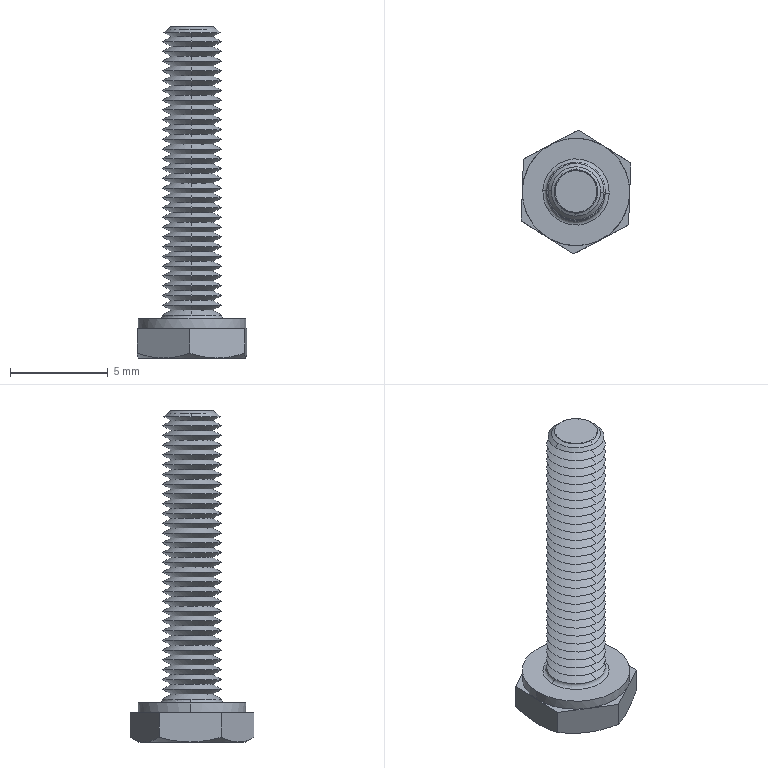Component | SolidWorks | GB_T5781-2000HexHeadBoltFullThreadGradeCM5_30-1 | 1 solid | 205 faces | volume 130 mm3 | cone 130 | cylinder 58 | plane 15 | torus 2 | commonest cylinder face diameters 3 x56 5.5 x2